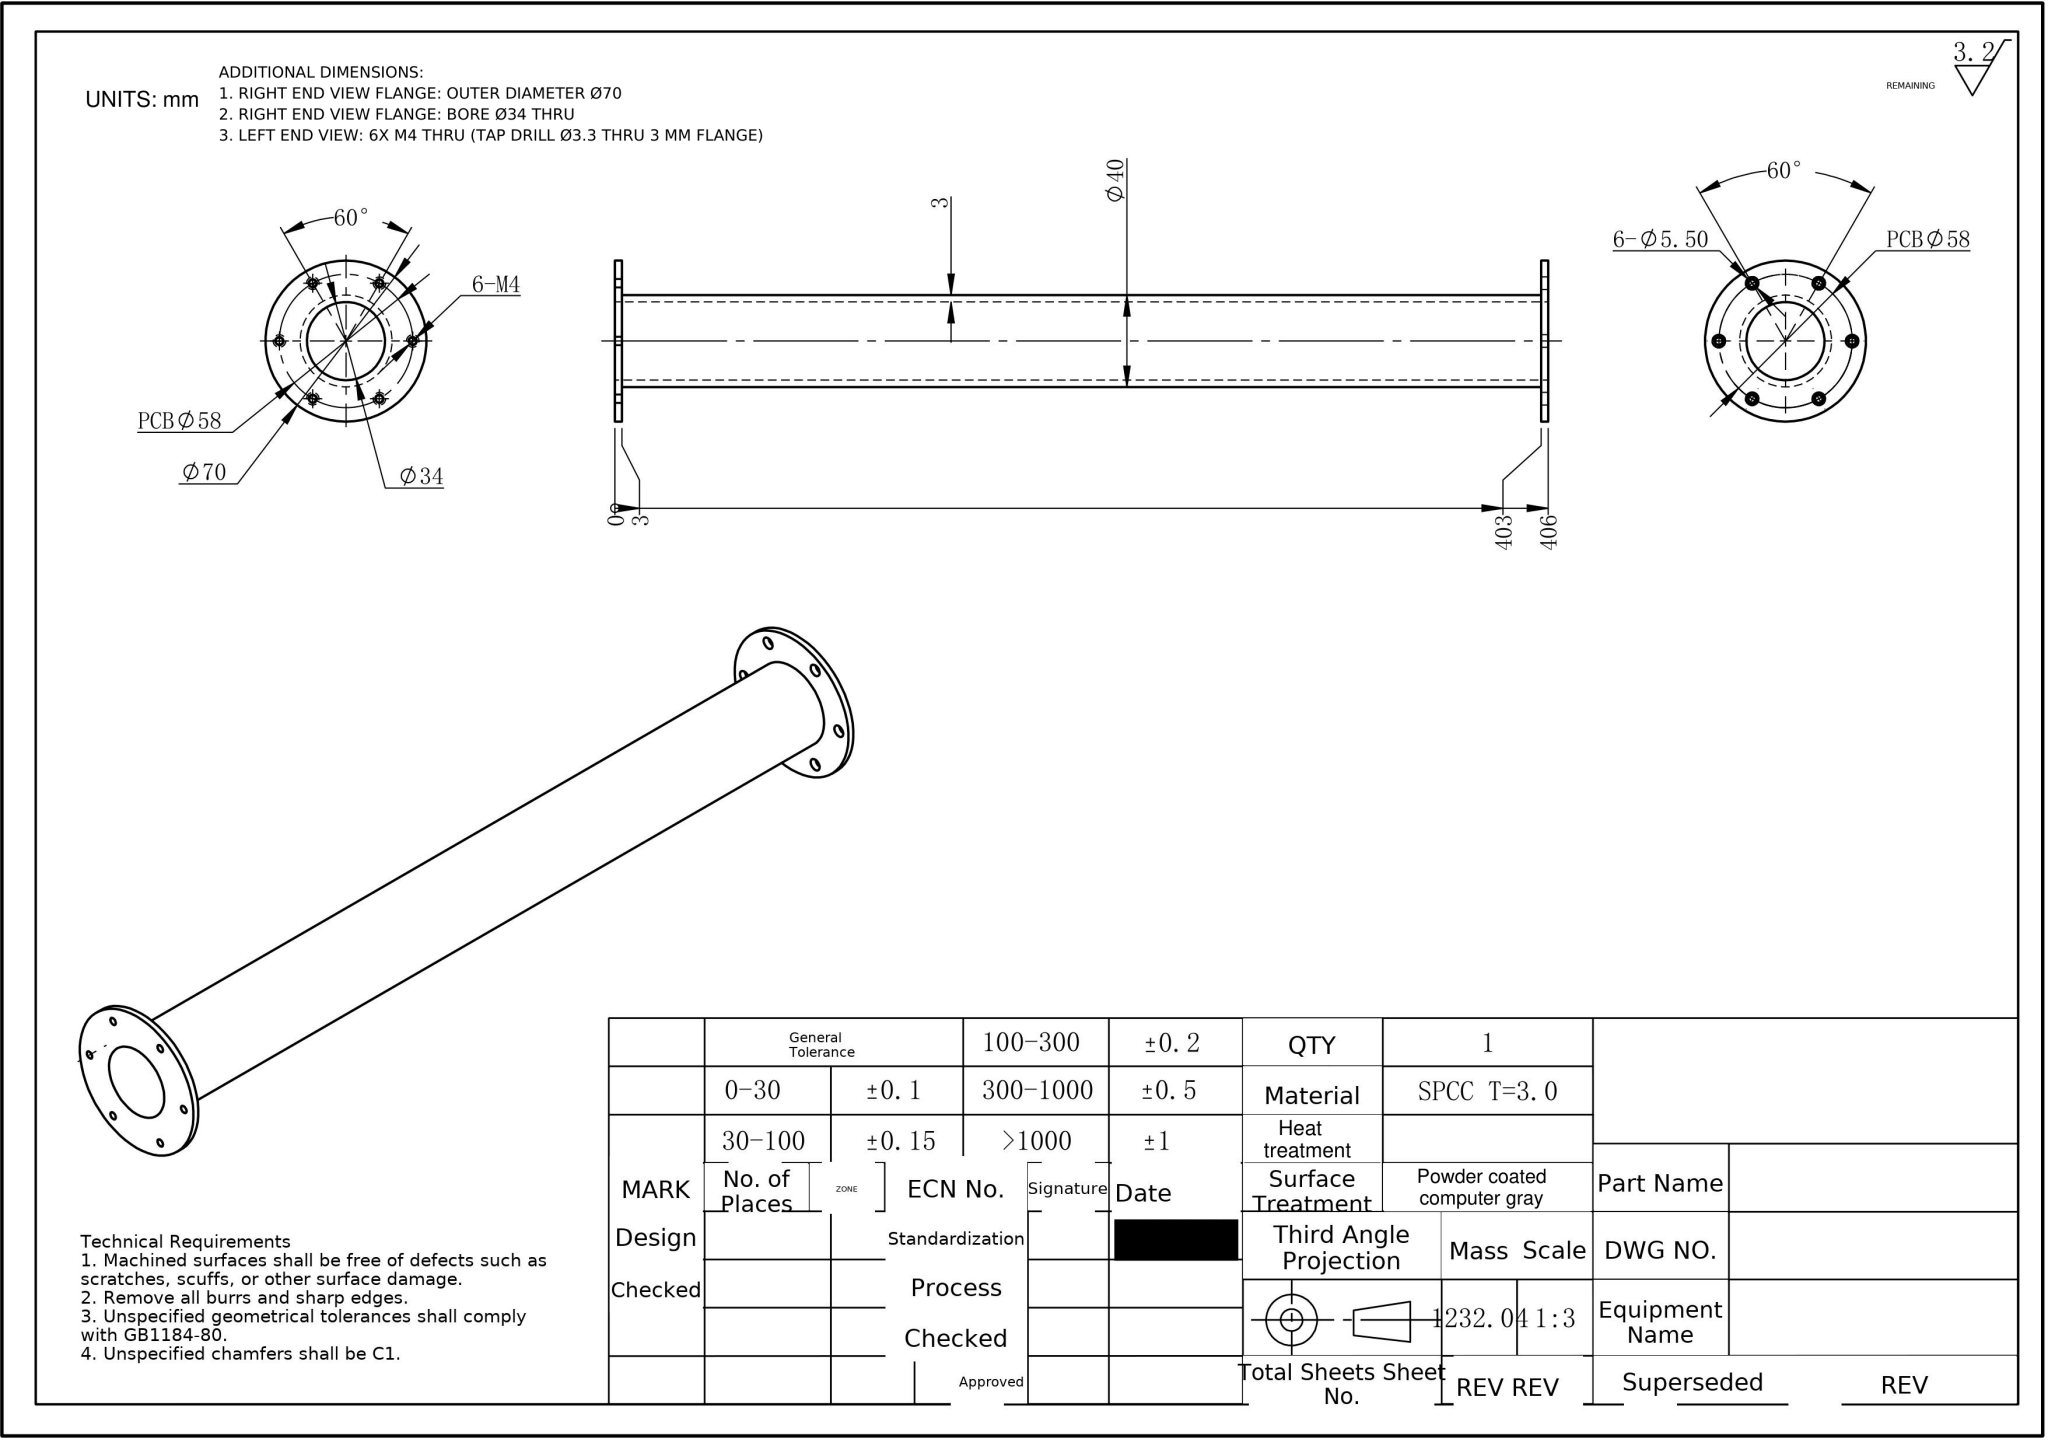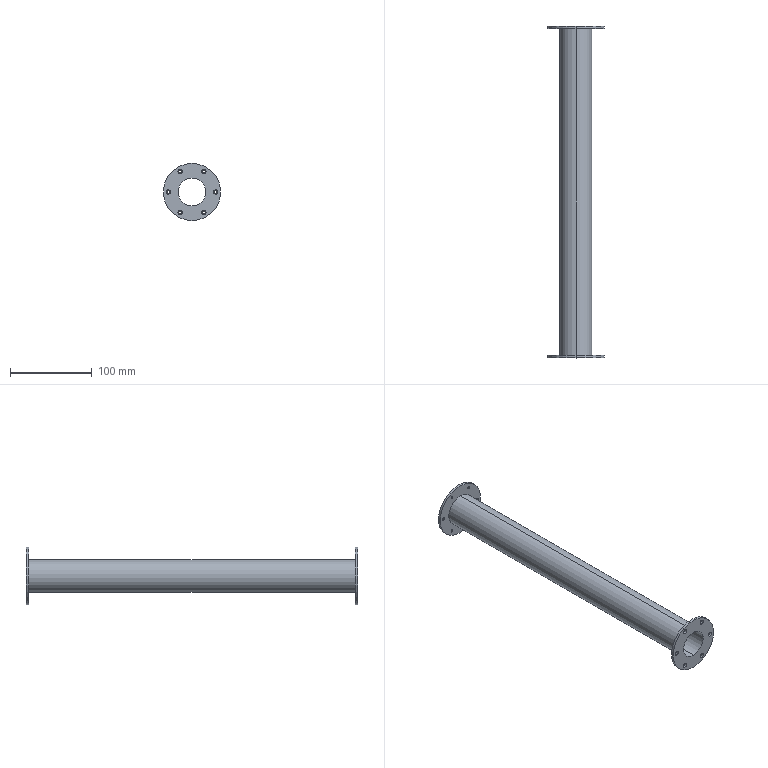Part | NX | mm | 1 solid | 36 faces | box 70 x 406 x 70 mm | volume 156548 mm3 | cylinder 32 | plane 4 | commonest cylinder face diameters 5.5 x12 3.3 x12 70 x4 34 x2 40 x2